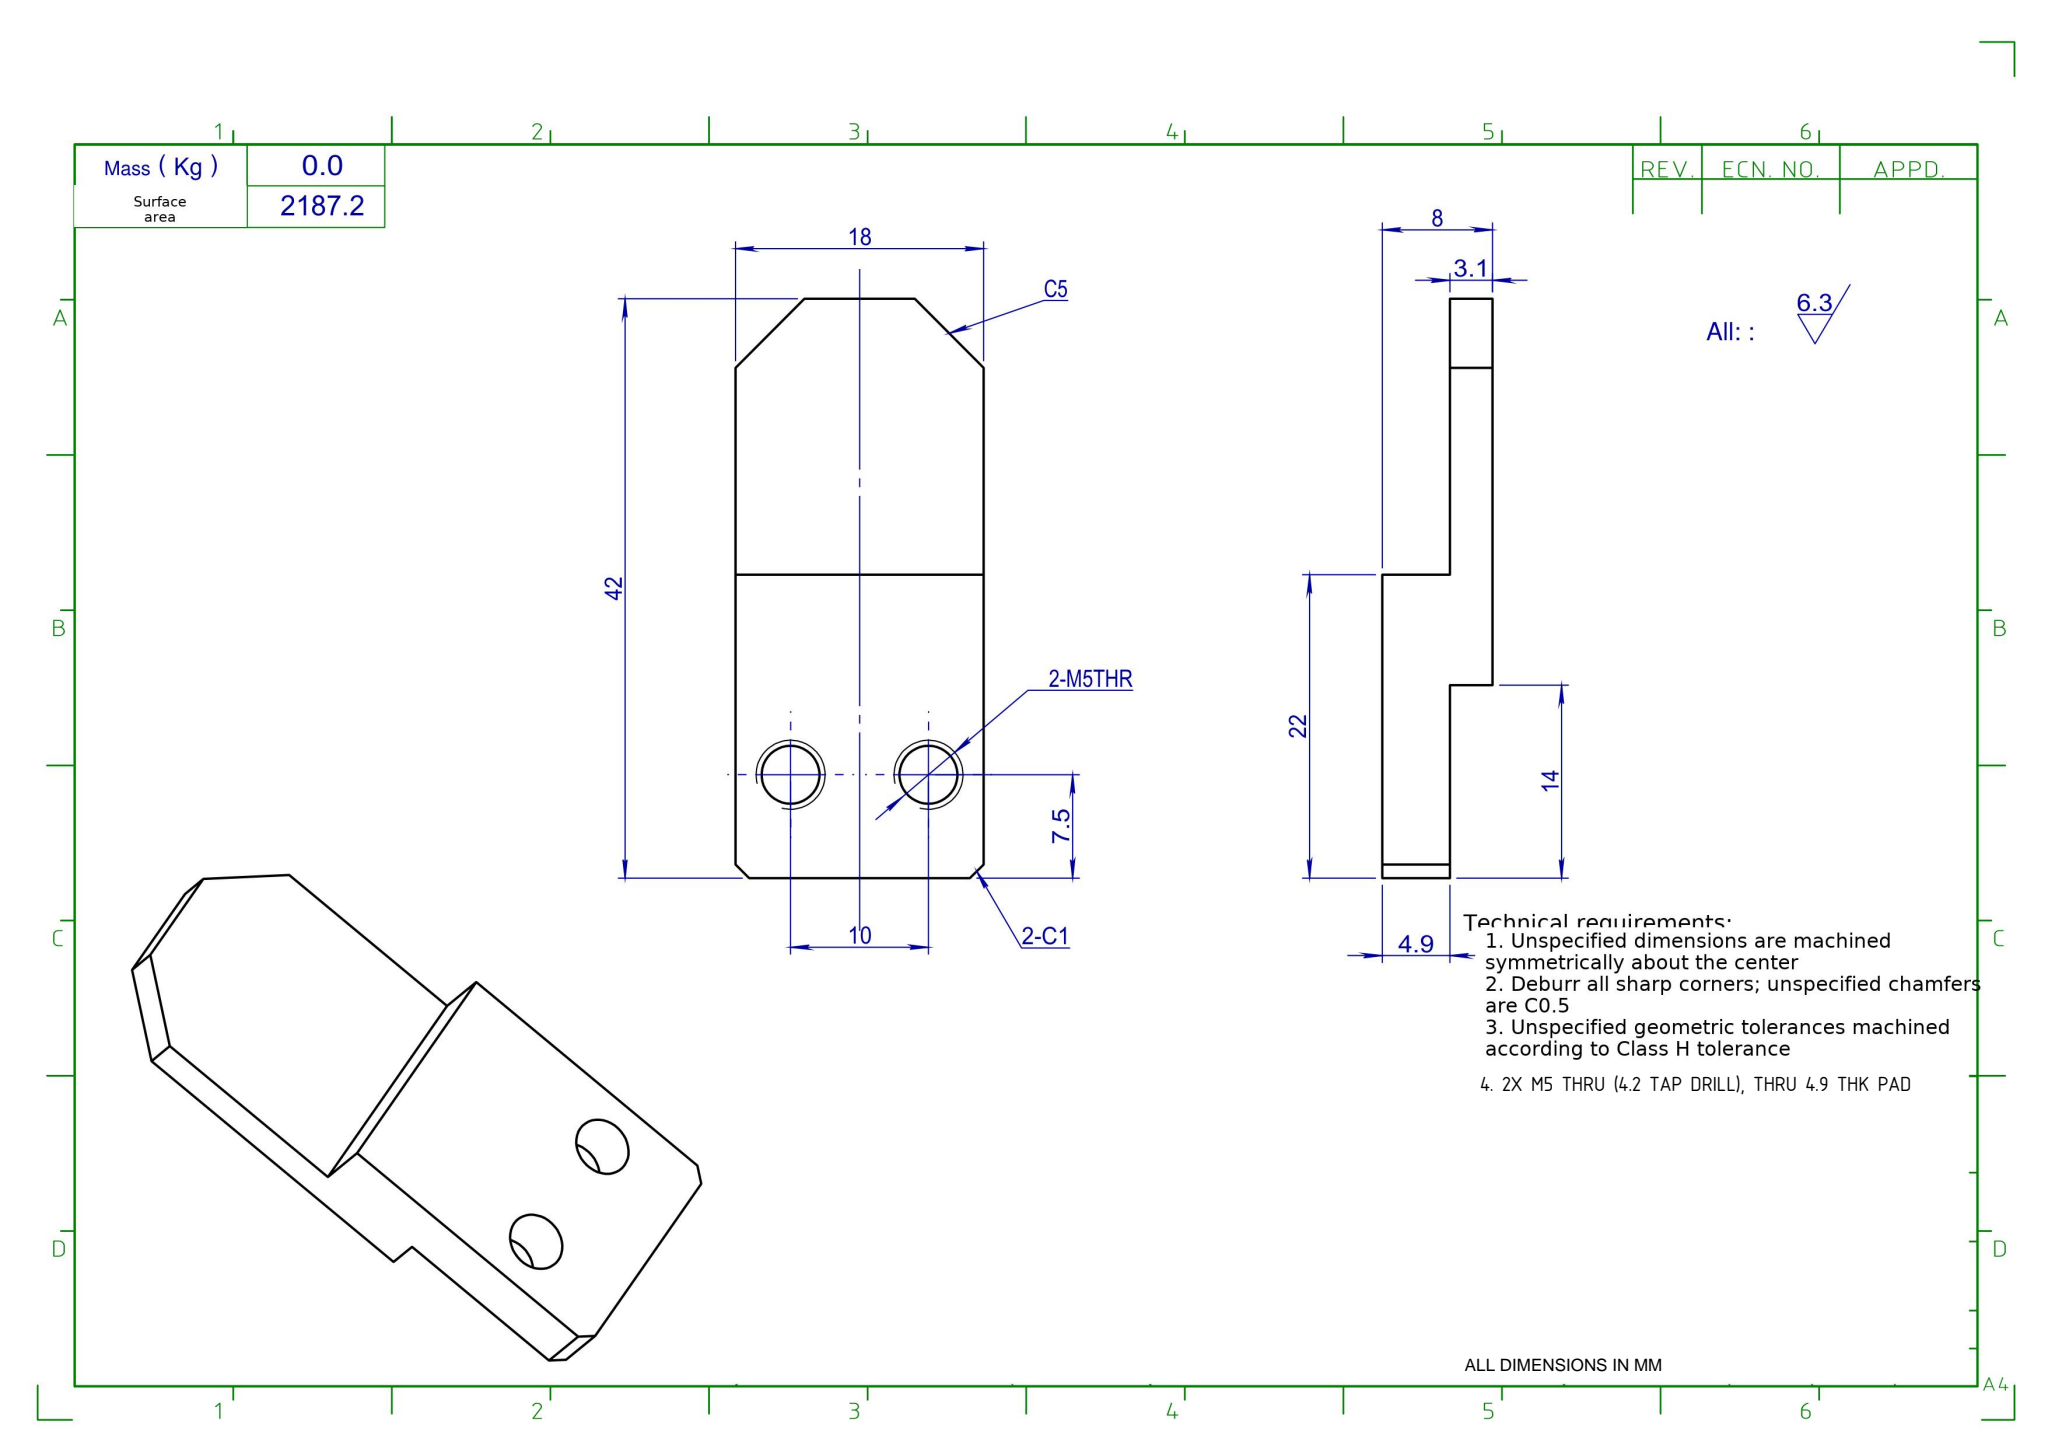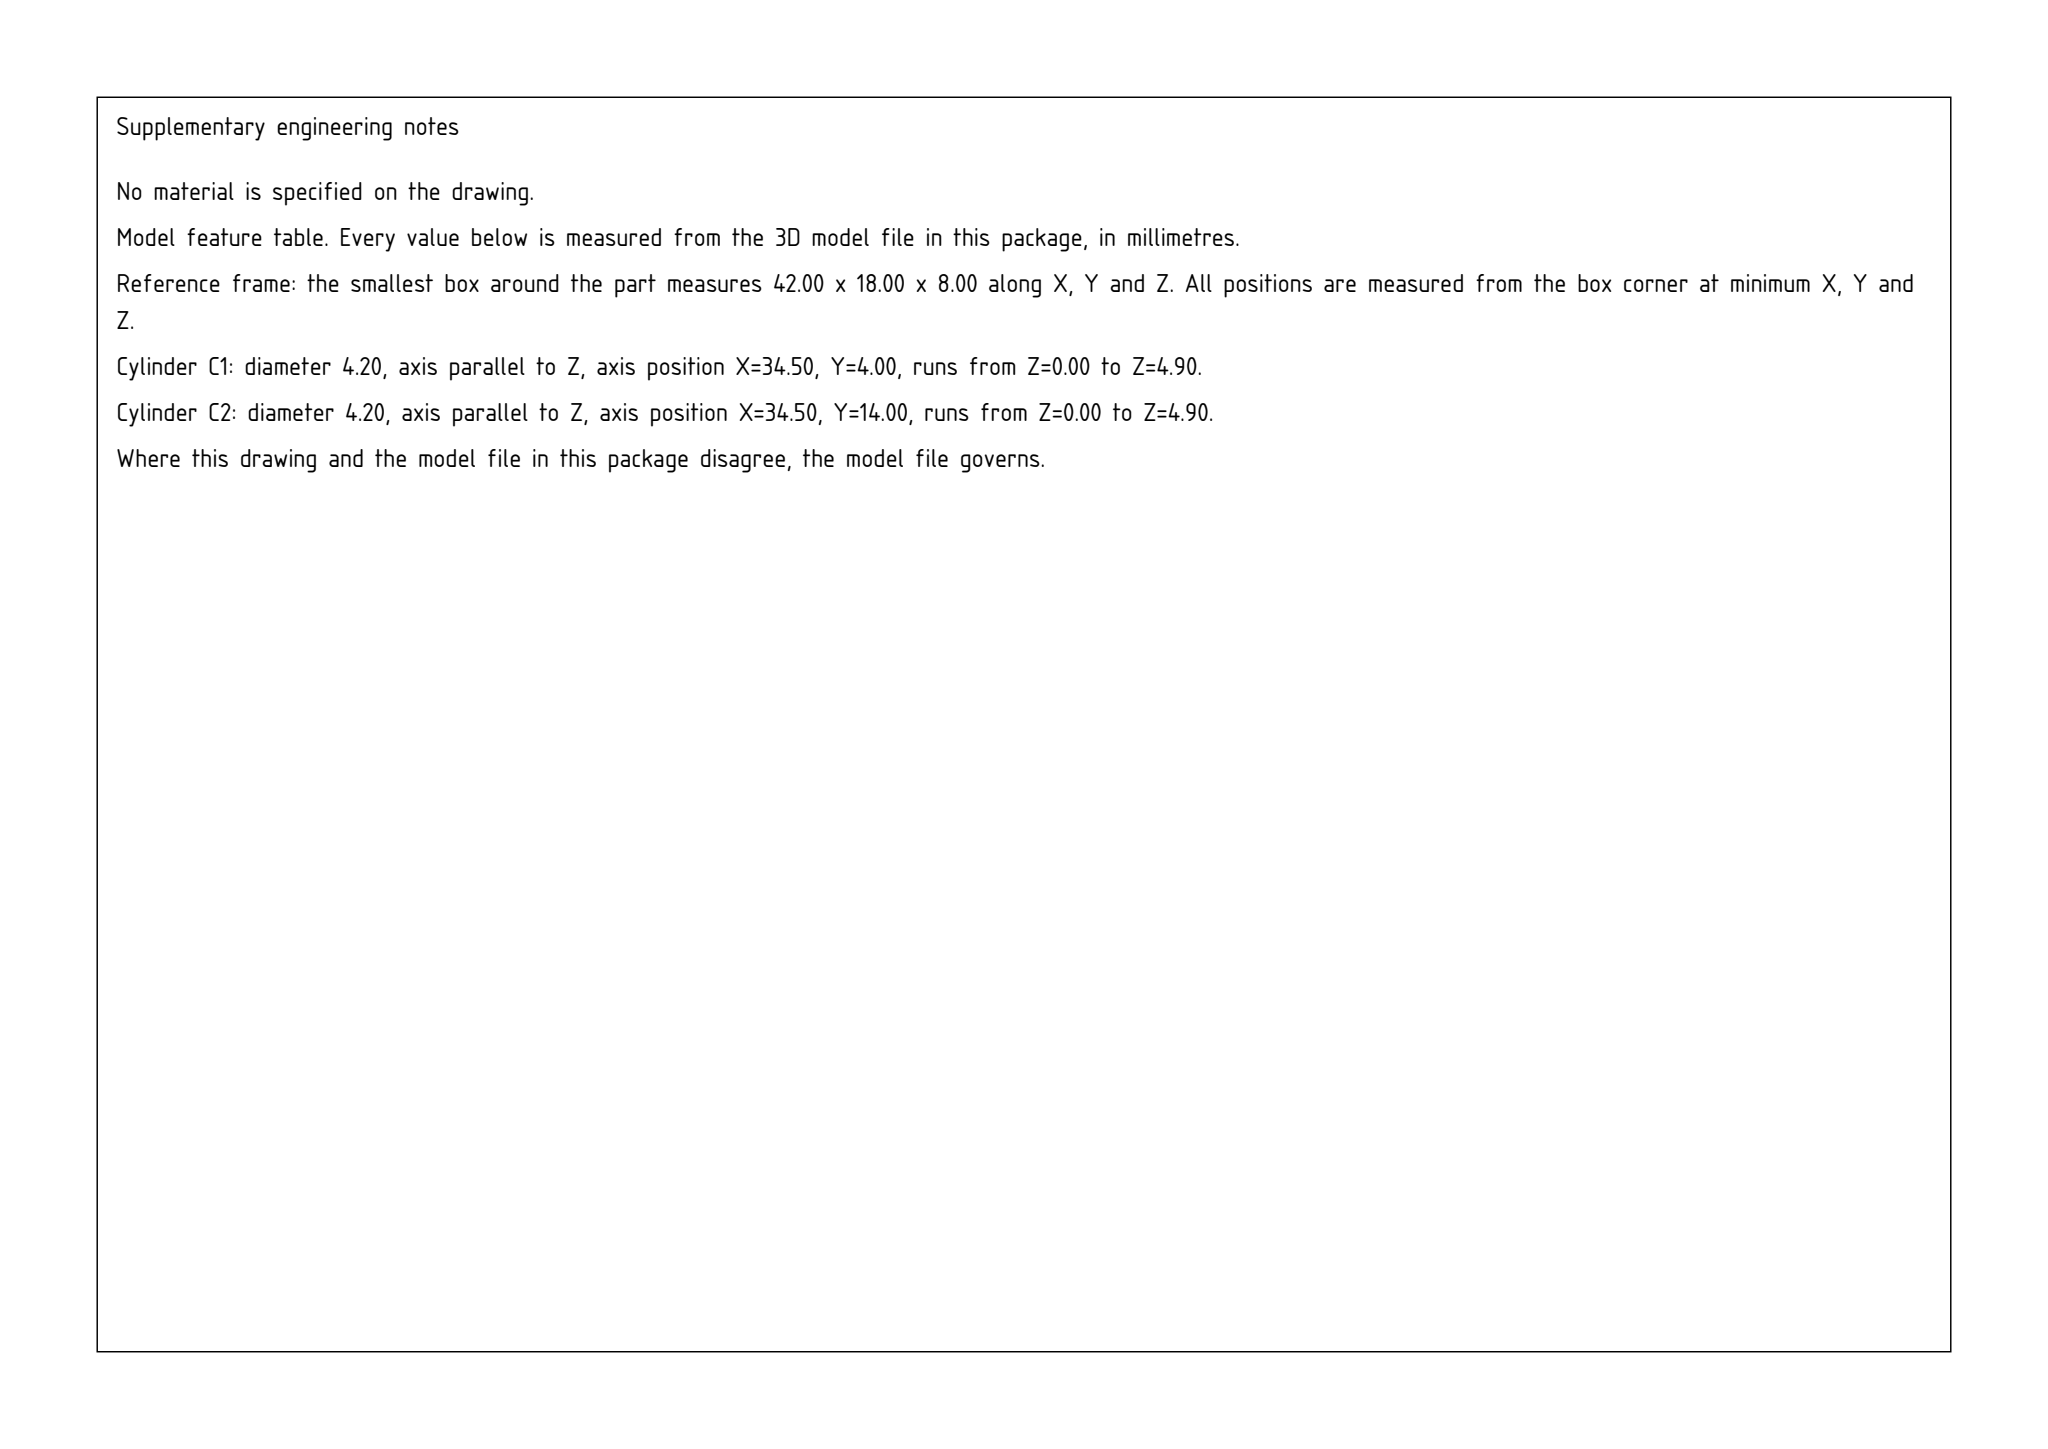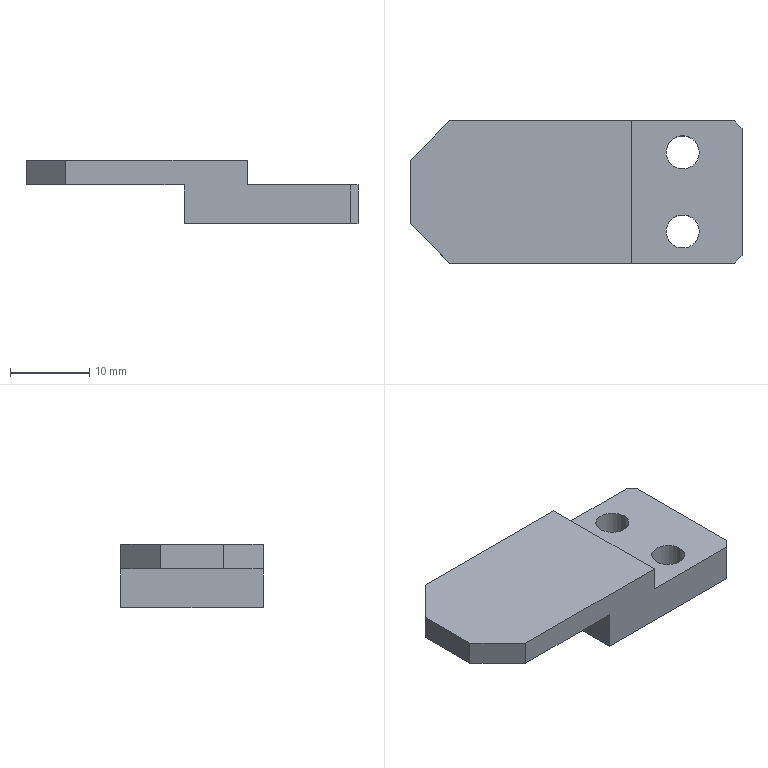Part | SolidWorks | mm | 1 solid | 18 faces | box 42 x 18 x 8 mm | volume 3285 mm3 | plane 14 | cylinder 4 | commonest cylinder face diameters 4.2 x4
Drawing notes:
2X M5 THRU (4.2 TAP DRILL), THRU 4.9 THK PAD | from the solid: cylinders: 2x hole/bore dia 4.2, axis z, from z=0.0 to z=4.9, full depth of 4.9 thk section (plane z=4.9 at x 28-42)
build123d program:
from build123d import *

# Parameters (mm, degrees)
SKETCH1_W             = 42
SKETCH1_H             = 18
BOSS_EXTRUDE1_DEPTH   = 4.9
SKETCH2_W             = 20
SKETCH2_H             = 5
CUT_EXTRUDE1_DEPTH    = 29.089
SKETCH3_W             = 28
SKETCH3_H             = 18
BOSS_EXTRUDE2_DEPTH   = 3.1
M5_TAPPED_HOLE1_D     = 4.2
M5_TAPPED_HOLE1_DEPTH = 13
M5_TAPPED_HOLE1_TIP   = 1.262
CHAMFER1_SIZE         = 5
CHAMFER2_SIZE         = 1


with BuildPart() as part:
    # Sketch1 → Boss-Extrude1 (new body)
    with BuildSketch(Plane.XY):
        Rectangle(SKETCH1_W, SKETCH1_H)
    extrude(amount=BOSS_EXTRUDE1_DEPTH)

    # Sketch2 → Cut-Extrude1 (cut, through all)
    with BuildSketch(Plane(origin=(0, 9, 0), x_dir=(1, 0, 0), z_dir=(0, 1, 0))):
        with Locations((-11, -2.5)):
            Rectangle(SKETCH2_W, SKETCH2_H)
    extrude(amount=-CUT_EXTRUDE1_DEPTH, mode=Mode.SUBTRACT)

    # Sketch3 → Boss-Extrude2 (add)
    with BuildSketch(Plane.XY.offset(4.9)):
        with Locations((-7, 0)):
            Rectangle(SKETCH3_W, SKETCH3_H)
    extrude(amount=BOSS_EXTRUDE2_DEPTH)

    # M5 Tapped Hole1
    with Locations(Plane.XY.offset(4.9)):
        with Locations((13.5, 5), (13.5, -5)):
            Hole(M5_TAPPED_HOLE1_D / 2, depth=M5_TAPPED_HOLE1_DEPTH)
            with Locations((0, 0, -(M5_TAPPED_HOLE1_DEPTH + M5_TAPPED_HOLE1_TIP / 2))):  # 118° drill point
                Cone(0, M5_TAPPED_HOLE1_D / 2, M5_TAPPED_HOLE1_TIP, mode=Mode.SUBTRACT)

    # Chamfer1
    chamfer1_edges = [part.edges().sort_by_distance(p)[0] for p in [
        (-21, 9, 6.45),
        (-21, -9, 6.45),
    ]]
    chamfer(chamfer1_edges, length=CHAMFER1_SIZE)

    # Chamfer2
    chamfer2_edges = [part.edges().sort_by_distance(p)[0] for p in [
        (21, -9, 2.45),
        (21, 9, 2.45),
    ]]
    chamfer(chamfer2_edges, length=CHAMFER2_SIZE)


solid = part.part
STEP:
#1=CARTESIAN_POINT('',(11.4,5.,0.));
#2=VERTEX_POINT('',#1);
#3=CARTESIAN_POINT('',(15.6,5.,0.));
#4=VERTEX_POINT('',#3);
#5=CARTESIAN_POINT('',(13.5,5.,0.));
#6=DIRECTION('',(0.,0.,1.));
#7=DIRECTION('',(1.,0.,0.));
#8=AXIS2_PLACEMENT_3D('',#5,#6,#7);
#9=CIRCLE('',#8,2.1);
#10=EDGE_CURVE('',#2,#4,#9,.T.);
#11=ORIENTED_EDGE('',*,*,#10,.F.);
#12=CARTESIAN_POINT('',(11.4,5.,4.9));
#13=VERTEX_POINT('',#12);
#14=CARTESIAN_POINT('',(11.4,5.,4.9));
#15=DIRECTION('',(0.,0.,1.));
#16=VECTOR('',#15,1000.);
#17=LINE('',#14,#16);
#18=EDGE_CURVE('',#2,#13,#17,.T.);
#19=ORIENTED_EDGE('',*,*,#18,.T.);
#20=CARTESIAN_POINT('',(15.6,5.,4.9));
#21=VERTEX_POINT('',#20);
#22=CARTESIAN_POINT('',(13.5,5.,4.9));
#23=DIRECTION('',(0.,0.,1.));
#24=DIRECTION('',(1.,0.,0.));
#25=AXIS2_PLACEMENT_3D('',#22,#23,#24);
#26=CIRCLE('',#25,2.1);
#27=EDGE_CURVE('',#13,#21,#26,.T.);
#28=ORIENTED_EDGE('',*,*,#27,.T.);
#29=CARTESIAN_POINT('',(15.6,5.,4.9));
#30=DIRECTION('',(0.,0.,1.));
#31=VECTOR('',#30,1000.);
#32=LINE('',#29,#31);
#33=EDGE_CURVE('',#4,#21,#32,.T.);
#34=ORIENTED_EDGE('',*,*,#33,.F.);
#35=EDGE_LOOP('',(#11,#19,#28,#34));
#36=FACE_OUTER_BOUND('',#35,.T.);
#37=CARTESIAN_POINT('',(13.5,5.,4.9));
#38=DIRECTION('',(0.,0.,1.));
#39=DIRECTION('',(1.,0.,0.));
#40=AXIS2_PLACEMENT_3D('',#37,#38,#39);
#41=CYLINDRICAL_SURFACE('',#40,2.1);
#42=ADVANCED_FACE('',(#36),#41,.F.);
#43=CARTESIAN_POINT('',(11.4,-5.,0.));
#44=VERTEX_POINT('',#43);
#45=CARTESIAN_POINT('',(15.6,-5.,0.));
#46=VERTEX_POINT('',#45);
#47=CARTESIAN_POINT('',(13.5,-5.,0.));
#48=DIRECTION('',(0.,0.,1.));
#49=DIRECTION('',(1.,0.,0.));
#50=AXIS2_PLACEMENT_3D('',#47,#48,#49);
#51=CIRCLE('',#50,2.1);
#52=EDGE_CURVE('',#44,#46,#51,.T.);
#53=ORIENTED_EDGE('',*,*,#52,.F.);
#54=CARTESIAN_POINT('',(11.4,-5.,4.9));
#55=VERTEX_POINT('',#54);
#56=CARTESIAN_POINT('',(11.4,-5.,4.9));
#57=DIRECTION('',(0.,0.,1.));
#58=VECTOR('',#57,1000.);
#59=LINE('',#56,#58);
#60=EDGE_CURVE('',#44,#55,#59,.T.);
#61=ORIENTED_EDGE('',*,*,#60,.T.);
#62=CARTESIAN_POINT('',(15.6,-5.,4.9));
#63=VERTEX_POINT('',#62);
#64=CARTESIAN_POINT('',(13.5,-5.,4.9));
#65=DIRECTION('',(0.,0.,1.));
#66=DIRECTION('',(1.,0.,0.));
#67=AXIS2_PLACEMENT_3D('',#64,#65,#66);
#68=CIRCLE('',#67,2.1);
#69=EDGE_CURVE('',#55,#63,#68,.T.);
#70=ORIENTED_EDGE('',*,*,#69,.T.);
#71=CARTESIAN_POINT('',(15.6,-5.,4.9));
#72=DIRECTION('',(0.,0.,1.));
#73=VECTOR('',#72,1000.);
#74=LINE('',#71,#73);
#75=EDGE_CURVE('',#46,#63,#74,.T.);
#76=ORIENTED_EDGE('',*,*,#75,.F.);
#77=EDGE_LOOP('',(#53,#61,#70,#76));
#78=FACE_OUTER_BOUND('',#77,.T.);
#79=CARTESIAN_POINT('',(13.5,-5.,4.9));
#80=DIRECTION('',(0.,0.,1.));
#81=DIRECTION('',(1.,0.,0.));
#82=AXIS2_PLACEMENT_3D('',#79,#80,#81);
#83=CYLINDRICAL_SURFACE('',#82,2.1);
#84=ADVANCED_FACE('',(#78),#83,.F.);
#85=CARTESIAN_POINT('',(-1.,-9.,0.));
#86=VERTEX_POINT('',#85);
#87=CARTESIAN_POINT('',(20.,-9.,0.));
#88=VERTEX_POINT('',#87);
#89=CARTESIAN_POINT('',(21.,-9.,0.));
#90=DIRECTION('',(1.,0.,0.));
#91=VECTOR('',#90,1000.);
#92=LINE('',#89,#91);
#93=EDGE_CURVE('',#86,#88,#92,.T.);
#94=ORIENTED_EDGE('',*,*,#93,.T.);
#95=CARTESIAN_POINT('',(20.,-9.,4.9));
#96=VERTEX_POINT('',#95);
#97=CARTESIAN_POINT('',(20.,-9.,4.9));
#98=DIRECTION('',(0.,0.,1.));
#99=VECTOR('',#98,1000.);
#100=LINE('',#97,#99);
#101=EDGE_CURVE('',#88,#96,#100,.T.);
#102=ORIENTED_EDGE('',*,*,#101,.T.);
#103=CARTESIAN_POINT('',(7.,-9.,4.9));
#104=VERTEX_POINT('',#103);
#105=CARTESIAN_POINT('',(21.,-9.,4.9));
#106=DIRECTION('',(1.,0.,0.));
#107=VECTOR('',#106,1000.);
#108=LINE('',#105,#107);
#109=EDGE_CURVE('',#104,#96,#108,.T.);
#110=ORIENTED_EDGE('',*,*,#109,.F.);
#111=CARTESIAN_POINT('',(7.,-9.,8.));
#112=VERTEX_POINT('',#111);
#113=CARTESIAN_POINT('',(7.,-9.,8.));
#114=DIRECTION('',(0.,0.,-1.));
#115=VECTOR('',#114,1000.);
#116=LINE('',#113,#115);
#117=EDGE_CURVE('',#112,#104,#116,.T.);
#118=ORIENTED_EDGE('',*,*,#117,.F.);
#119=CARTESIAN_POINT('',(-16.,-9.,8.));
#120=VERTEX_POINT('',#119);
#121=CARTESIAN_POINT('',(-21.,-9.,8.));
#122=DIRECTION('',(1.,0.,0.));
#123=VECTOR('',#122,1000.);
#124=LINE('',#121,#123);
#125=EDGE_CURVE('',#120,#112,#124,.T.);
#126=ORIENTED_EDGE('',*,*,#125,.F.);
#127=CARTESIAN_POINT('',(-16.,-9.,4.9));
#128=VERTEX_POINT('',#127);
#129=CARTESIAN_POINT('',(-16.,-9.,4.9));
#130=DIRECTION('',(0.,0.,-1.));
#131=VECTOR('',#130,1000.);
#132=LINE('',#129,#131);
#133=EDGE_CURVE('',#120,#128,#132,.T.);
#134=ORIENTED_EDGE('',*,*,#133,.T.);
#135=CARTESIAN_POINT('',(-1.,-9.,4.9));
#136=VERTEX_POINT('',#135);
#137=CARTESIAN_POINT('',(-21.,-9.,4.9));
#138=DIRECTION('',(1.,0.,0.));
#139=VECTOR('',#138,1000.);
#140=LINE('',#137,#139);
#141=EDGE_CURVE('',#128,#136,#140,.T.);
#142=ORIENTED_EDGE('',*,*,#141,.T.);
#143=CARTESIAN_POINT('',(-1.,-9.,0.));
#144=DIRECTION('',(0.,0.,-1.));
#145=VECTOR('',#144,1000.);
#146=LINE('',#143,#145);
#147=EDGE_CURVE('',#136,#86,#146,.T.);
#148=ORIENTED_EDGE('',*,*,#147,.T.);
#149=EDGE_LOOP('',(#94,#102,#110,#118,#126,#134,#142,#148));
#150=FACE_OUTER_BOUND('',#149,.T.);
#151=CARTESIAN_POINT('',(21.,-9.,4.9));
#152=DIRECTION('',(-0.,1.,0.));
#153=DIRECTION('',(-1.,-0.,0.));
#154=AXIS2_PLACEMENT_3D('',#151,#152,#153);
#155=PLANE('',#154);
#156=ADVANCED_FACE('',(#150),#155,.F.);
#157=CARTESIAN_POINT('',(21.,-8.,4.9));
#158=VERTEX_POINT('',#157);
#159=CARTESIAN_POINT('',(21.,8.,4.9));
#160=VERTEX_POINT('',#159);
#161=CARTESIAN_POINT('',(21.,-9.,4.9));
#162=DIRECTION('',(0.,1.,0.));
#163=VECTOR('',#162,1000.);
#164=LINE('',#161,#163);
#165=EDGE_CURVE('',#158,#160,#164,.T.);
#166=ORIENTED_EDGE('',*,*,#165,.F.);
#167=CARTESIAN_POINT('',(21.,-8.,0.));
#168=VERTEX_POINT('',#167);
#169=CARTESIAN_POINT('',(21.,-8.,4.9));
#170=DIRECTION('',(0.,0.,-1.));
#171=VECTOR('',#170,1000.);
#172=LINE('',#169,#171);
#173=EDGE_CURVE('',#158,#168,#172,.T.);
#174=ORIENTED_EDGE('',*,*,#173,.T.);
#175=CARTESIAN_POINT('',(21.,8.,0.));
#176=VERTEX_POINT('',#175);
#177=CARTESIAN_POINT('',(21.,-9.,0.));
#178=DIRECTION('',(0.,1.,0.));
#179=VECTOR('',#178,1000.);
#180=LINE('',#177,#179);
#181=EDGE_CURVE('',#168,#176,#180,.T.);
#182=ORIENTED_EDGE('',*,*,#181,.T.);
#183=CARTESIAN_POINT('',(21.,8.,4.9));
#184=DIRECTION('',(0.,0.,1.));
#185=VECTOR('',#184,1000.);
#186=LINE('',#183,#185);
#187=EDGE_CURVE('',#176,#160,#186,.T.);
#188=ORIENTED_EDGE('',*,*,#187,.T.);
#189=EDGE_LOOP('',(#166,#174,#182,#188));
#190=FACE_OUTER_BOUND('',#189,.T.);
#191=CARTESIAN_POINT('',(21.,-9.,4.9));
#192=DIRECTION('',(-1.,0.,0.));
#193=DIRECTION('',(0.,0.,1.));
#194=AXIS2_PLACEMENT_3D('',#191,#192,#193);
#195=PLANE('',#194);
#196=ADVANCED_FACE('',(#190),#195,.F.);
#197=CARTESIAN_POINT('',(20.,9.,4.9));
#198=VERTEX_POINT('',#197);
#199=CARTESIAN_POINT('',(7.,9.,4.9));
#200=VERTEX_POINT('',#199);
#201=CARTESIAN_POINT('',(21.,9.,4.9));
#202=DIRECTION('',(-1.,-0.,0.));
#203=VECTOR('',#202,1000.);
#204=LINE('',#201,#203);
#205=EDGE_CURVE('',#198,#200,#204,.T.);
#206=ORIENTED_EDGE('',*,*,#205,.F.);
#207=CARTESIAN_POINT('',(20.,9.,0.));
#208=VERTEX_POINT('',#207);
#209=CARTESIAN_POINT('',(20.,9.,4.9));
#210=DIRECTION('',(0.,0.,-1.));
#211=VECTOR('',#210,1000.);
#212=LINE('',#209,#211);
#213=EDGE_CURVE('',#198,#208,#212,.T.);
#214=ORIENTED_EDGE('',*,*,#213,.T.);
#215=CARTESIAN_POINT('',(-1.,9.,0.));
#216=VERTEX_POINT('',#215);
#217=CARTESIAN_POINT('',(21.,9.,0.));
#218=DIRECTION('',(-1.,-0.,0.));
#219=VECTOR('',#218,1000.);
#220=LINE('',#217,#219);
#221=EDGE_CURVE('',#208,#216,#220,.T.);
#222=ORIENTED_EDGE('',*,*,#221,.T.);
#223=CARTESIAN_POINT('',(-1.,9.,4.9));
#224=VERTEX_POINT('',#223);
#225=CARTESIAN_POINT('',(-1.,9.,0.));
#226=DIRECTION('',(0.,0.,-1.));
#227=VECTOR('',#226,1000.);
#228=LINE('',#225,#227);
#229=EDGE_CURVE('',#224,#216,#228,.T.);
#230=ORIENTED_EDGE('',*,*,#229,.F.);
#231=CARTESIAN_POINT('',(-16.,9.,4.9));
#232=VERTEX_POINT('',#231);
#233=CARTESIAN_POINT('',(-21.,9.,4.9));
#234=DIRECTION('',(-1.,0.,0.));
#235=VECTOR('',#234,1000.);
#236=LINE('',#233,#235);
#237=EDGE_CURVE('',#224,#232,#236,.T.);
#238=ORIENTED_EDGE('',*,*,#237,.T.);
#239=CARTESIAN_POINT('',(-16.,9.,8.));
#240=VERTEX_POINT('',#239);
#241=CARTESIAN_POINT('',(-16.,9.,4.9));
#242=DIRECTION('',(0.,0.,1.));
#243=VECTOR('',#242,1000.);
#244=LINE('',#241,#243);
#245=EDGE_CURVE('',#232,#240,#244,.T.);
#246=ORIENTED_EDGE('',*,*,#245,.T.);
#247=CARTESIAN_POINT('',(7.,9.,8.));
#248=VERTEX_POINT('',#247);
#249=CARTESIAN_POINT('',(-21.,9.,8.));
#250=DIRECTION('',(-1.,0.,0.));
#251=VECTOR('',#250,1000.);
#252=LINE('',#249,#251);
#253=EDGE_CURVE('',#248,#240,#252,.T.);
#254=ORIENTED_EDGE('',*,*,#253,.F.);
#255=CARTESIAN_POINT('',(7.,9.,8.));
#256=DIRECTION('',(0.,0.,-1.));
#257=VECTOR('',#256,1000.);
#258=LINE('',#255,#257);
#259=EDGE_CURVE('',#248,#200,#258,.T.);
#260=ORIENTED_EDGE('',*,*,#259,.T.);
#261=EDGE_LOOP('',(#206,#214,#222,#230,#238,#246,#254,#260));
#262=FACE_OUTER_BOUND('',#261,.T.);
#263=CARTESIAN_POINT('',(21.,9.,4.9));
#264=DIRECTION('',(0.,-1.,0.));
#265=DIRECTION('',(1.,0.,0.));
#266=AXIS2_PLACEMENT_3D('',#263,#264,#265);
#267=PLANE('',#266);
#268=ADVANCED_FACE('',(#262),#267,.F.);
#269=CARTESIAN_POINT('',(13.5,5.,4.9));
#270=DIRECTION('',(0.,0.,1.));
#271=DIRECTION('',(1.,0.,0.));
#272=AXIS2_PLACEMENT_3D('',#269,#270,#271);
#273=CIRCLE('',#272,2.1);
#274=EDGE_CURVE('',#21,#13,#273,.T.);
#275=ORIENTED_EDGE('',*,*,#274,.F.);
#276=ORIENTED_EDGE('',*,*,#27,.F.);
#277=EDGE_LOOP('',(#275,#276));
#278=FACE_BOUND('',#277,.T.);
#279=CARTESIAN_POINT('',(13.5,-5.,4.9));
#280=DIRECTION('',(0.,0.,1.));
#281=DIRECTION('',(1.,0.,0.));
#282=AXIS2_PLACEMENT_3D('',#279,#280,#281);
#283=CIRCLE('',#282,2.1);
#284=EDGE_CURVE('',#63,#55,#283,.T.);
#285=ORIENTED_EDGE('',*,*,#284,.F.);
#286=ORIENTED_EDGE('',*,*,#69,.F.);
#287=EDGE_LOOP('',(#285,#286));
#288=FACE_BOUND('',#287,.T.);
#289=ORIENTED_EDGE('',*,*,#109,.T.);
#290=CARTESIAN_POINT('',(14.5,-14.5,4.9));
#291=DIRECTION('',(0.7071,0.7071,0.));
#292=VECTOR('',#291,1000.);
#293=LINE('',#290,#292);
#294=EDGE_CURVE('',#96,#158,#293,.T.);
#295=ORIENTED_EDGE('',*,*,#294,.T.);
#296=ORIENTED_EDGE('',*,*,#165,.T.);
#297=CARTESIAN_POINT('',(14.5,14.5,4.9));
#298=DIRECTION('',(-0.7071,0.7071,0.));
#299=VECTOR('',#298,1000.);
#300=LINE('',#297,#299);
#301=EDGE_CURVE('',#160,#198,#300,.T.);
#302=ORIENTED_EDGE('',*,*,#301,.T.);
#303=ORIENTED_EDGE('',*,*,#205,.T.);
#304=CARTESIAN_POINT('',(7.,9.,4.9));
#305=DIRECTION('',(-0.,1.,0.));
#306=VECTOR('',#305,1000.);
#307=LINE('',#304,#306);
#308=EDGE_CURVE('',#104,#200,#307,.T.);
#309=ORIENTED_EDGE('',*,*,#308,.F.);
#310=EDGE_LOOP('',(#289,#295,#296,#302,#303,#309));
#311=FACE_OUTER_BOUND('',#310,.T.);
#312=CARTESIAN_POINT('',(0.,0.,4.9));
#313=DIRECTION('',(0.,0.,1.));
#314=DIRECTION('',(1.,0.,0.));
#315=AXIS2_PLACEMENT_3D('',#312,#313,#314);
#316=PLANE('',#315);
#317=ADVANCED_FACE('',(#278,#288,#311),#316,.T.);
#318=CARTESIAN_POINT('',(13.5,5.,0.));
#319=DIRECTION('',(0.,0.,1.));
#320=DIRECTION('',(1.,0.,0.));
#321=AXIS2_PLACEMENT_3D('',#318,#319,#320);
#322=CIRCLE('',#321,2.1);
#323=EDGE_CURVE('',#4,#2,#322,.T.);
#324=ORIENTED_EDGE('',*,*,#323,.T.);
#325=ORIENTED_EDGE('',*,*,#10,.T.);
#326=EDGE_LOOP('',(#324,#325));
#327=FACE_BOUND('',#326,.T.);
#328=CARTESIAN_POINT('',(13.5,-5.,0.));
#329=DIRECTION('',(0.,0.,1.));
#330=DIRECTION('',(1.,0.,0.));
#331=AXIS2_PLACEMENT_3D('',#328,#329,#330);
#332=CIRCLE('',#331,2.1);
#333=EDGE_CURVE('',#46,#44,#332,.T.);
#334=ORIENTED_EDGE('',*,*,#333,.T.);
#335=ORIENTED_EDGE('',*,*,#52,.T.);
#336=EDGE_LOOP('',(#334,#335));
#337=FACE_BOUND('',#336,.T.);
#338=ORIENTED_EDGE('',*,*,#181,.F.);
#339=CARTESIAN_POINT('',(21.,-8.,0.));
#340=DIRECTION('',(-0.7071,-0.7071,0.));
#341=VECTOR('',#340,1000.);
#342=LINE('',#339,#341);
#343=EDGE_CURVE('',#168,#88,#342,.T.);
#344=ORIENTED_EDGE('',*,*,#343,.T.);
#345=ORIENTED_EDGE('',*,*,#93,.F.);
#346=CARTESIAN_POINT('',(-1.,-9.,0.));
#347=DIRECTION('',(-0.,1.,0.));
#348=VECTOR('',#347,1000.);
#349=LINE('',#346,#348);
#350=EDGE_CURVE('',#86,#216,#349,.T.);
#351=ORIENTED_EDGE('',*,*,#350,.T.);
#352=ORIENTED_EDGE('',*,*,#221,.F.);
#353=CARTESIAN_POINT('',(20.,9.,0.));
#354=DIRECTION('',(0.7071,-0.7071,0.));
#355=VECTOR('',#354,1000.);
#356=LINE('',#353,#355);
#357=EDGE_CURVE('',#208,#176,#356,.T.);
#358=ORIENTED_EDGE('',*,*,#357,.T.);
#359=EDGE_LOOP('',(#338,#344,#345,#351,#352,#358));
#360=FACE_OUTER_BOUND('',#359,.T.);
#361=CARTESIAN_POINT('',(0.,0.,0.));
#362=DIRECTION('',(0.,0.,1.));
#363=DIRECTION('',(1.,0.,0.));
#364=AXIS2_PLACEMENT_3D('',#361,#362,#363);
#365=PLANE('',#364);
#366=ADVANCED_FACE('',(#327,#337,#360),#365,.F.);
#367=CARTESIAN_POINT('',(-1.,-0.,4.9));
#368=DIRECTION('',(-0.,1.,0.));
#369=VECTOR('',#368,1000.);
#370=LINE('',#367,#369);
#371=EDGE_CURVE('',#136,#224,#370,.T.);
#372=ORIENTED_EDGE('',*,*,#371,.T.);
#373=ORIENTED_EDGE('',*,*,#229,.T.);
#374=ORIENTED_EDGE('',*,*,#350,.F.);
#375=ORIENTED_EDGE('',*,*,#147,.F.);
#376=EDGE_LOOP('',(#372,#373,#374,#375));
#377=FACE_OUTER_BOUND('',#376,.T.);
#378=CARTESIAN_POINT('',(-1.,-9.,0.));
#379=DIRECTION('',(1.,0.,0.));
#380=DIRECTION('',(-0.,1.,0.));
#381=AXIS2_PLACEMENT_3D('',#378,#379,#380);
#382=PLANE('',#381);
#383=ADVANCED_FACE('',(#377),#382,.F.);
#384=CARTESIAN_POINT('',(-21.,4.,8.));
#385=VERTEX_POINT('',#384);
#386=CARTESIAN_POINT('',(-21.,-4.,8.));
#387=VERTEX_POINT('',#386);
#388=CARTESIAN_POINT('',(-21.,9.,8.));
#389=DIRECTION('',(0.,-1.,0.));
#390=VECTOR('',#389,1000.);
#391=LINE('',#388,#390);
#392=EDGE_CURVE('',#385,#387,#391,.T.);
#393=ORIENTED_EDGE('',*,*,#392,.F.);
#394=CARTESIAN_POINT('',(-21.,4.,4.9));
#395=VERTEX_POINT('',#394);
#396=CARTESIAN_POINT('',(-21.,4.,8.));
#397=DIRECTION('',(0.,0.,-1.));
#398=VECTOR('',#397,1000.);
#399=LINE('',#396,#398);
#400=EDGE_CURVE('',#385,#395,#399,.T.);
#401=ORIENTED_EDGE('',*,*,#400,.T.);
#402=CARTESIAN_POINT('',(-21.,-4.,4.9));
#403=VERTEX_POINT('',#402);
#404=CARTESIAN_POINT('',(-21.,9.,4.9));
#405=DIRECTION('',(0.,-1.,0.));
#406=VECTOR('',#405,1000.);
#407=LINE('',#404,#406);
#408=EDGE_CURVE('',#395,#403,#407,.T.);
#409=ORIENTED_EDGE('',*,*,#408,.T.);
#410=CARTESIAN_POINT('',(-21.,-4.,8.));
#411=DIRECTION('',(0.,0.,1.));
#412=VECTOR('',#411,1000.);
#413=LINE('',#410,#412);
#414=EDGE_CURVE('',#403,#387,#413,.T.);
#415=ORIENTED_EDGE('',*,*,#414,.T.);
#416=EDGE_LOOP('',(#393,#401,#409,#415));
#417=FACE_OUTER_BOUND('',#416,.T.);
#418=CARTESIAN_POINT('',(-21.,9.,8.));
#419=DIRECTION('',(1.,0.,0.));
#420=DIRECTION('',(-0.,1.,0.));
#421=AXIS2_PLACEMENT_3D('',#418,#419,#420);
#422=PLANE('',#421);
#423=ADVANCED_FACE('',(#417),#422,.F.);
#424=ORIENTED_EDGE('',*,*,#308,.T.);
#425=ORIENTED_EDGE('',*,*,#259,.F.);
#426=CARTESIAN_POINT('',(7.,9.,8.));
#427=DIRECTION('',(-0.,1.,0.));
#428=VECTOR('',#427,1000.);
#429=LINE('',#426,#428);
#430=EDGE_CURVE('',#112,#248,#429,.T.);
#431=ORIENTED_EDGE('',*,*,#430,.F.);
#432=ORIENTED_EDGE('',*,*,#117,.T.);
#433=EDGE_LOOP('',(#424,#425,#431,#432));
#434=FACE_OUTER_BOUND('',#433,.T.);
#435=CARTESIAN_POINT('',(7.,9.,8.));
#436=DIRECTION('',(-1.,-0.,0.));
#437=DIRECTION('',(0.,-1.,0.));
#438=AXIS2_PLACEMENT_3D('',#435,#436,#437);
#439=PLANE('',#438);
#440=ADVANCED_FACE('',(#434),#439,.F.);
#441=ORIENTED_EDGE('',*,*,#253,.T.);
#442=CARTESIAN_POINT('',(-12.5,12.5,8.));
#443=DIRECTION('',(-0.7071,-0.7071,0.));
#444=VECTOR('',#443,1000.);
#445=LINE('',#442,#444);
#446=EDGE_CURVE('',#240,#385,#445,.T.);
#447=ORIENTED_EDGE('',*,*,#446,.T.);
#448=ORIENTED_EDGE('',*,*,#392,.T.);
#449=CARTESIAN_POINT('',(-12.5,-12.5,8.));
#450=DIRECTION('',(0.7071,-0.7071,0.));
#451=VECTOR('',#450,1000.);
#452=LINE('',#449,#451);
#453=EDGE_CURVE('',#387,#120,#452,.T.);
#454=ORIENTED_EDGE('',*,*,#453,.T.);
#455=ORIENTED_EDGE('',*,*,#125,.T.);
#456=ORIENTED_EDGE('',*,*,#430,.T.);
#457=EDGE_LOOP('',(#441,#447,#448,#454,#455,#456));
#458=FACE_OUTER_BOUND('',#457,.T.);
#459=CARTESIAN_POINT('',(0.,0.,8.));
#460=DIRECTION('',(0.,0.,1.));
#461=DIRECTION('',(1.,0.,0.));
#462=AXIS2_PLACEMENT_3D('',#459,#460,#461);
#463=PLANE('',#462);
#464=ADVANCED_FACE('',(#458),#463,.T.);
#465=ORIENTED_EDGE('',*,*,#408,.F.);
#466=CARTESIAN_POINT('',(-21.,4.,4.9));
#467=DIRECTION('',(0.7071,0.7071,0.));
#468=VECTOR('',#467,1000.);
#469=LINE('',#466,#468);
#470=EDGE_CURVE('',#395,#232,#469,.T.);
#471=ORIENTED_EDGE('',*,*,#470,.T.);
#472=ORIENTED_EDGE('',*,*,#237,.F.);
#473=ORIENTED_EDGE('',*,*,#371,.F.);
#474=ORIENTED_EDGE('',*,*,#141,.F.);
#475=CARTESIAN_POINT('',(-16.,-9.,4.9));
#476=DIRECTION('',(-0.7071,0.7071,0.));
#477=VECTOR('',#476,1000.);
#478=LINE('',#475,#477);
#479=EDGE_CURVE('',#128,#403,#478,.T.);
#480=ORIENTED_EDGE('',*,*,#479,.T.);
#481=EDGE_LOOP('',(#465,#471,#472,#473,#474,#480));
#482=FACE_OUTER_BOUND('',#481,.T.);
#483=CARTESIAN_POINT('',(0.,0.,4.9));
#484=DIRECTION('',(0.,0.,1.));
#485=DIRECTION('',(1.,0.,0.));
#486=AXIS2_PLACEMENT_3D('',#483,#484,#485);
#487=PLANE('',#486);
#488=ADVANCED_FACE('',(#482),#487,.F.);
#489=ORIENTED_EDGE('',*,*,#60,.F.);
#490=ORIENTED_EDGE('',*,*,#333,.F.);
#491=ORIENTED_EDGE('',*,*,#75,.T.);
#492=ORIENTED_EDGE('',*,*,#284,.T.);
#493=EDGE_LOOP('',(#489,#490,#491,#492));
#494=FACE_OUTER_BOUND('',#493,.T.);
#495=CARTESIAN_POINT('',(13.5,-5.,4.9));
#496=DIRECTION('',(0.,0.,1.));
#497=DIRECTION('',(1.,0.,0.));
#498=AXIS2_PLACEMENT_3D('',#495,#496,#497);
#499=CYLINDRICAL_SURFACE('',#498,2.1);
#500=ADVANCED_FACE('',(#494),#499,.F.);
#501=ORIENTED_EDGE('',*,*,#18,.F.);
#502=ORIENTED_EDGE('',*,*,#323,.F.);
#503=ORIENTED_EDGE('',*,*,#33,.T.);
#504=ORIENTED_EDGE('',*,*,#274,.T.);
#505=EDGE_LOOP('',(#501,#502,#503,#504));
#506=FACE_OUTER_BOUND('',#505,.T.);
#507=CARTESIAN_POINT('',(13.5,5.,4.9));
#508=DIRECTION('',(0.,0.,1.));
#509=DIRECTION('',(1.,0.,0.));
#510=AXIS2_PLACEMENT_3D('',#507,#508,#509);
#511=CYLINDRICAL_SURFACE('',#510,2.1);
#512=ADVANCED_FACE('',(#506),#511,.F.);
#513=ORIENTED_EDGE('',*,*,#446,.F.);
#514=ORIENTED_EDGE('',*,*,#245,.F.);
#515=ORIENTED_EDGE('',*,*,#470,.F.);
#516=ORIENTED_EDGE('',*,*,#400,.F.);
#517=EDGE_LOOP('',(#513,#514,#515,#516));
#518=FACE_OUTER_BOUND('',#517,.T.);
#519=CARTESIAN_POINT('',(-21.,4.,8.));
#520=DIRECTION('',(0.7071,-0.7071,0.));
#521=DIRECTION('',(0.,0.,-1.));
#522=AXIS2_PLACEMENT_3D('',#519,#520,#521);
#523=PLANE('',#522);
#524=ADVANCED_FACE('',(#518),#523,.F.);
#525=ORIENTED_EDGE('',*,*,#453,.F.);
#526=ORIENTED_EDGE('',*,*,#414,.F.);
#527=ORIENTED_EDGE('',*,*,#479,.F.);
#528=ORIENTED_EDGE('',*,*,#133,.F.);
#529=EDGE_LOOP('',(#525,#526,#527,#528));
#530=FACE_OUTER_BOUND('',#529,.T.);
#531=CARTESIAN_POINT('',(-16.,-9.,4.9));
#532=DIRECTION('',(0.7071,0.7071,0.));
#533=DIRECTION('',(0.,0.,-1.));
#534=AXIS2_PLACEMENT_3D('',#531,#532,#533);
#535=PLANE('',#534);
#536=ADVANCED_FACE('',(#530),#535,.F.);
#537=ORIENTED_EDGE('',*,*,#294,.F.);
#538=ORIENTED_EDGE('',*,*,#101,.F.);
#539=ORIENTED_EDGE('',*,*,#343,.F.);
#540=ORIENTED_EDGE('',*,*,#173,.F.);
#541=EDGE_LOOP('',(#537,#538,#539,#540));
#542=FACE_OUTER_BOUND('',#541,.T.);
#543=CARTESIAN_POINT('',(21.,-8.,4.9));
#544=DIRECTION('',(-0.7071,0.7071,0.));
#545=DIRECTION('',(0.,0.,-1.));
#546=AXIS2_PLACEMENT_3D('',#543,#544,#545);
#547=PLANE('',#546);
#548=ADVANCED_FACE('',(#542),#547,.F.);
#549=ORIENTED_EDGE('',*,*,#301,.F.);
#550=ORIENTED_EDGE('',*,*,#187,.F.);
#551=ORIENTED_EDGE('',*,*,#357,.F.);
#552=ORIENTED_EDGE('',*,*,#213,.F.);
#553=EDGE_LOOP('',(#549,#550,#551,#552));
#554=FACE_OUTER_BOUND('',#553,.T.);
#555=CARTESIAN_POINT('',(20.,9.,4.9));
#556=DIRECTION('',(-0.7071,-0.7071,0.));
#557=DIRECTION('',(0.,0.,-1.));
#558=AXIS2_PLACEMENT_3D('',#555,#556,#557);
#559=PLANE('',#558);
#560=ADVANCED_FACE('',(#554),#559,.F.);
#561=CLOSED_SHELL('',(#42,#84,#156,#196,#268,#317,#366,#383,#423,#440,#464,#488,#500,#512,#524,#536,#548,#560));
#562=MANIFOLD_SOLID_BREP('',#561);
#563=CARTESIAN_POINT('',(0.,0.,0.));
#564=DIRECTION('',(0.,0.,1.));
#565=DIRECTION('',(1.,0.,0.));
#566=AXIS2_PLACEMENT_3D('',#563,#564,#565);
#567=(LENGTH_UNIT()NAMED_UNIT(*)SI_UNIT(.MILLI.,.METRE.));
#568=UNCERTAINTY_MEASURE_WITH_UNIT(LENGTH_MEASURE(0.00001),#567,'','');
#569=(NAMED_UNIT(*)PLANE_ANGLE_UNIT()SI_UNIT($,.RADIAN.));
#570=(NAMED_UNIT(*)SI_UNIT($,.STERADIAN.)SOLID_ANGLE_UNIT());
#571=(GEOMETRIC_REPRESENTATION_CONTEXT(3)GLOBAL_UNCERTAINTY_ASSIGNED_CONTEXT((#568))GLOBAL_UNIT_ASSIGNED_CONTEXT((#567,#569,#570))REPRESENTATION_CONTEXT('',''));
#572=ADVANCED_BREP_SHAPE_REPRESENTATION('',(#562,#566),#571);